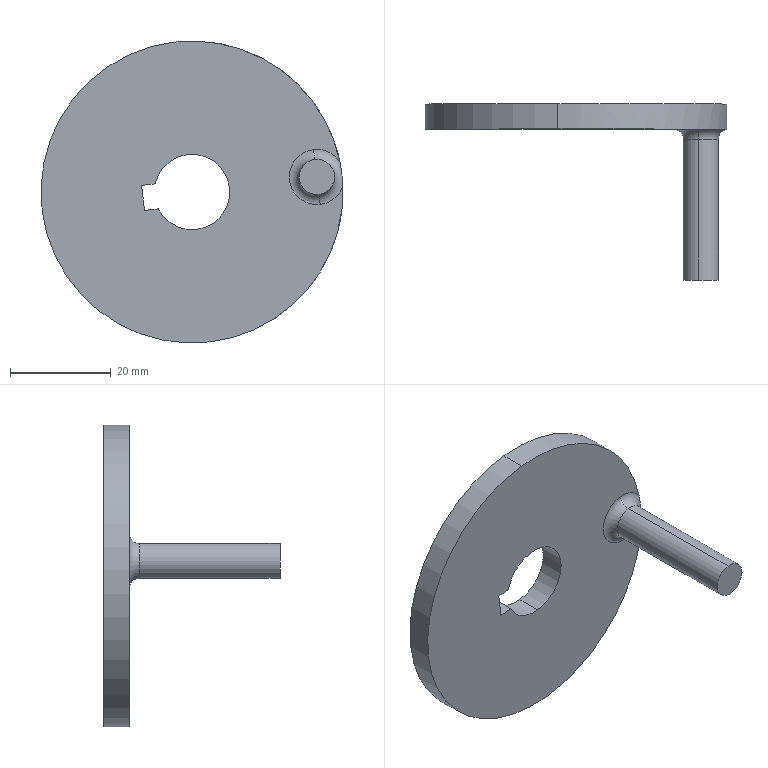Component | SolidWorks | CrankshaftOne-2_NewCrank-1 | 1 solid | 15 faces | box 60 x 35 x 60 mm | volume 14368 mm3 | cylinder 7 | plane 6 | torus 2 | commonest cylinder face diameters 15 x3 7 x2 60 x2 | material AISI 1045 Steel, Cold Drawn
STEP:
#1=COLOUR_RGB('',0.7922,0.8196,0.9333);
#2=FILL_AREA_STYLE_COLOUR('',#1);
#3=FILL_AREA_STYLE('',(#2));
#4=SURFACE_STYLE_FILL_AREA(#3);
#5=SURFACE_SIDE_STYLE('',(#4));
#6=SURFACE_STYLE_USAGE(.BOTH.,#5);
#7=PRESENTATION_STYLE_ASSIGNMENT((#6));
#8=CARTESIAN_POINT('',(1.263,0.7191,-6.574));
#9=VERTEX_POINT('',#8);
#10=CARTESIAN_POINT('',(1.23,0.7191,-6.301));
#11=VERTEX_POINT('',#10);
#12=CARTESIAN_POINT('',(1.247,0.7191,-6.438));
#13=DIRECTION('',(-0.,-1.,-0.));
#14=DIRECTION('',(0.1196,0.,-0.9928));
#15=AXIS2_PLACEMENT_3D('',#12,#13,#14);
#16=CIRCLE('',#15,0.1378);
#17=EDGE_CURVE('',#9,#11,#16,.T.);
#18=ORIENTED_EDGE('',*,*,#17,.F.);
#19=CARTESIAN_POINT('',(1.263,1.821,-6.574));
#20=VERTEX_POINT('',#19);
#21=CARTESIAN_POINT('',(1.263,0.7191,-6.574));
#22=DIRECTION('',(0.,1.,0.));
#23=VECTOR('',#22,39.37);
#24=LINE('',#21,#23);
#25=EDGE_CURVE('',#9,#20,#24,.T.);
#26=ORIENTED_EDGE('',*,*,#25,.T.);
#27=CARTESIAN_POINT('',(1.23,1.821,-6.301));
#28=VERTEX_POINT('',#27);
#29=CARTESIAN_POINT('',(1.247,1.821,-6.438));
#30=DIRECTION('',(-0.,-1.,-0.));
#31=DIRECTION('',(-0.1196,0.,0.9928));
#32=AXIS2_PLACEMENT_3D('',#29,#30,#31);
#33=CIRCLE('',#32,0.1378);
#34=EDGE_CURVE('',#20,#28,#33,.T.);
#35=ORIENTED_EDGE('',*,*,#34,.T.);
#36=CARTESIAN_POINT('',(1.23,0.7191,-6.301));
#37=DIRECTION('',(0.,1.,0.));
#38=VECTOR('',#37,39.37);
#39=LINE('',#36,#38);
#40=EDGE_CURVE('',#11,#28,#39,.T.);
#41=ORIENTED_EDGE('',*,*,#40,.F.);
#42=EDGE_LOOP('',(#18,#26,#35,#41));
#43=FACE_OUTER_BOUND('',#42,.T.);
#44=CARTESIAN_POINT('',(1.247,0.7191,-6.438));
#45=DIRECTION('',(0.,1.,0.));
#46=DIRECTION('',(-0.1196,0.,0.9928));
#47=AXIS2_PLACEMENT_3D('',#44,#45,#46);
#48=CYLINDRICAL_SURFACE('',#47,0.1378);
#49=ADVANCED_FACE('',(#43),#48,.T.);
#50=CARTESIAN_POINT('',(0.1282,2.097,-5.383));
#51=VERTEX_POINT('',#50);
#52=CARTESIAN_POINT('',(0.4108,2.097,-7.728));
#53=VERTEX_POINT('',#52);
#54=CARTESIAN_POINT('',(0.2695,2.097,-6.555));
#55=DIRECTION('',(0.,1.,0.));
#56=DIRECTION('',(-0.1196,0.,0.9928));
#57=AXIS2_PLACEMENT_3D('',#54,#55,#56);
#58=CIRCLE('',#57,1.181);
#59=EDGE_CURVE('',#51,#53,#58,.T.);
#60=ORIENTED_EDGE('',*,*,#59,.F.);
#61=CARTESIAN_POINT('',(0.1282,1.9,-5.383));
#62=VERTEX_POINT('',#61);
#63=CARTESIAN_POINT('',(0.1282,2.097,-5.383));
#64=DIRECTION('',(-0.,-1.,-0.));
#65=VECTOR('',#64,39.37);
#66=LINE('',#63,#65);
#67=EDGE_CURVE('',#51,#62,#66,.T.);
#68=ORIENTED_EDGE('',*,*,#67,.T.);
#69=CARTESIAN_POINT('',(1.426,1.9,-6.317));
#70=VERTEX_POINT('',#69);
#71=CARTESIAN_POINT('',(0.2695,1.9,-6.555));
#72=DIRECTION('',(0.,1.,0.));
#73=DIRECTION('',(-0.1196,0.,0.9928));
#74=AXIS2_PLACEMENT_3D('',#71,#72,#73);
#75=CIRCLE('',#74,1.181);
#76=EDGE_CURVE('',#62,#70,#75,.T.);
#77=ORIENTED_EDGE('',*,*,#76,.T.);
#78=CARTESIAN_POINT('',(1.45,1.9,-6.513));
#79=VERTEX_POINT('',#78);
#80=CARTESIAN_POINT('',(1.426,1.9,-6.317));
#81=CARTESIAN_POINT('',(1.43,1.9,-6.333));
#82=CARTESIAN_POINT('',(1.433,1.9,-6.349));
#83=CARTESIAN_POINT('',(1.438,1.898,-6.381));
#84=CARTESIAN_POINT('',(1.44,1.898,-6.398));
#85=CARTESIAN_POINT('',(1.444,1.898,-6.43));
#86=CARTESIAN_POINT('',(1.446,1.898,-6.447));
#87=CARTESIAN_POINT('',(1.448,1.9,-6.48));
#88=CARTESIAN_POINT('',(1.449,1.9,-6.496));
#89=CARTESIAN_POINT('',(1.45,1.9,-6.513));
#90=B_SPLINE_CURVE_WITH_KNOTS('',3,(#80,#81,#82,#83,#84,#85,#86,#87,#88,#89),.UNSPECIFIED.,.F.,.F.,(4,2,2,2,4),(0.,0.001254,0.002508,0.003762,0.005016),.UNSPECIFIED.);
#91=EDGE_CURVE('',#70,#79,#90,.T.);
#92=ORIENTED_EDGE('',*,*,#91,.T.);
#93=CARTESIAN_POINT('',(0.4108,1.9,-7.728));
#94=VERTEX_POINT('',#93);
#95=CARTESIAN_POINT('',(0.2695,1.9,-6.555));
#96=DIRECTION('',(0.,1.,0.));
#97=DIRECTION('',(-0.1196,0.,0.9928));
#98=AXIS2_PLACEMENT_3D('',#95,#96,#97);
#99=CIRCLE('',#98,1.181);
#100=EDGE_CURVE('',#79,#94,#99,.T.);
#101=ORIENTED_EDGE('',*,*,#100,.T.);
#102=CARTESIAN_POINT('',(0.4108,2.097,-7.728));
#103=DIRECTION('',(-0.,-1.,-0.));
#104=VECTOR('',#103,39.37);
#105=LINE('',#102,#104);
#106=EDGE_CURVE('',#53,#94,#105,.T.);
#107=ORIENTED_EDGE('',*,*,#106,.F.);
#108=EDGE_LOOP('',(#60,#68,#77,#92,#101,#107));
#109=FACE_OUTER_BOUND('',#108,.T.);
#110=CARTESIAN_POINT('',(0.2695,2.097,-6.555));
#111=DIRECTION('',(-0.,-1.,-0.));
#112=DIRECTION('',(0.1196,0.,-0.9928));
#113=AXIS2_PLACEMENT_3D('',#110,#111,#112);
#114=CYLINDRICAL_SURFACE('',#113,1.181);
#115=ADVANCED_FACE('',(#109),#114,.T.);
#116=CARTESIAN_POINT('',(-0.01865,2.097,-6.491));
#117=VERTEX_POINT('',#116);
#118=CARTESIAN_POINT('',(0.2342,2.097,-6.262));
#119=VERTEX_POINT('',#118);
#120=CARTESIAN_POINT('',(0.2695,2.097,-6.555));
#121=DIRECTION('',(0.,1.,0.));
#122=DIRECTION('',(-0.1196,0.,0.9928));
#123=AXIS2_PLACEMENT_3D('',#120,#121,#122);
#124=CIRCLE('',#123,0.2953);
#125=EDGE_CURVE('',#117,#119,#124,.T.);
#126=ORIENTED_EDGE('',*,*,#125,.T.);
#127=CARTESIAN_POINT('',(0.2342,1.9,-6.262));
#128=VERTEX_POINT('',#127);
#129=CARTESIAN_POINT('',(0.2342,2.097,-6.262));
#130=DIRECTION('',(-0.,-1.,-0.));
#131=VECTOR('',#130,39.37);
#132=LINE('',#129,#131);
#133=EDGE_CURVE('',#119,#128,#132,.T.);
#134=ORIENTED_EDGE('',*,*,#133,.T.);
#135=CARTESIAN_POINT('',(-0.01865,1.9,-6.491));
#136=VERTEX_POINT('',#135);
#137=CARTESIAN_POINT('',(0.2695,1.9,-6.555));
#138=DIRECTION('',(0.,1.,0.));
#139=DIRECTION('',(-0.1196,0.,0.9928));
#140=AXIS2_PLACEMENT_3D('',#137,#138,#139);
#141=CIRCLE('',#140,0.2953);
#142=EDGE_CURVE('',#136,#128,#141,.T.);
#143=ORIENTED_EDGE('',*,*,#142,.F.);
#144=CARTESIAN_POINT('',(-0.01865,2.097,-6.491));
#145=DIRECTION('',(-0.,-1.,-0.));
#146=VECTOR('',#145,39.37);
#147=LINE('',#144,#146);
#148=EDGE_CURVE('',#117,#136,#147,.T.);
#149=ORIENTED_EDGE('',*,*,#148,.F.);
#150=EDGE_LOOP('',(#126,#134,#143,#149));
#151=FACE_OUTER_BOUND('',#150,.T.);
#152=CARTESIAN_POINT('',(0.2695,2.097,-6.555));
#153=DIRECTION('',(-0.,-1.,-0.));
#154=DIRECTION('',(0.1196,0.,-0.9928));
#155=AXIS2_PLACEMENT_3D('',#152,#153,#154);
#156=CYLINDRICAL_SURFACE('',#155,0.2953);
#157=ADVANCED_FACE('',(#151),#156,.F.);
#158=ORIENTED_EDGE('',*,*,#133,.F.);
#159=CARTESIAN_POINT('',(0.3048,2.097,-6.849));
#160=VERTEX_POINT('',#159);
#161=CARTESIAN_POINT('',(0.2695,2.097,-6.555));
#162=DIRECTION('',(0.,1.,0.));
#163=DIRECTION('',(-0.1196,0.,0.9928));
#164=AXIS2_PLACEMENT_3D('',#161,#162,#163);
#165=CIRCLE('',#164,0.2953);
#166=EDGE_CURVE('',#119,#160,#165,.T.);
#167=ORIENTED_EDGE('',*,*,#166,.T.);
#168=CARTESIAN_POINT('',(0.3048,1.9,-6.849));
#169=VERTEX_POINT('',#168);
#170=CARTESIAN_POINT('',(0.3048,2.097,-6.849));
#171=DIRECTION('',(-0.,-1.,-0.));
#172=VECTOR('',#171,39.37);
#173=LINE('',#170,#172);
#174=EDGE_CURVE('',#160,#169,#173,.T.);
#175=ORIENTED_EDGE('',*,*,#174,.T.);
#176=CARTESIAN_POINT('',(0.2695,1.9,-6.555));
#177=DIRECTION('',(0.,1.,0.));
#178=DIRECTION('',(-0.1196,0.,0.9928));
#179=AXIS2_PLACEMENT_3D('',#176,#177,#178);
#180=CIRCLE('',#179,0.2953);
#181=EDGE_CURVE('',#128,#169,#180,.T.);
#182=ORIENTED_EDGE('',*,*,#181,.F.);
#183=EDGE_LOOP('',(#158,#167,#175,#182));
#184=FACE_OUTER_BOUND('',#183,.T.);
#185=CARTESIAN_POINT('',(0.2695,2.097,-6.555));
#186=DIRECTION('',(-0.,-1.,-0.));
#187=DIRECTION('',(0.1196,0.,-0.9928));
#188=AXIS2_PLACEMENT_3D('',#185,#186,#187);
#189=CYLINDRICAL_SURFACE('',#188,0.2953);
#190=ADVANCED_FACE('',(#184),#189,.F.);
#191=CARTESIAN_POINT('',(1.273,1.9,-6.653));
#192=VERTEX_POINT('',#191);
#193=CARTESIAN_POINT('',(1.221,1.9,-6.223));
#194=VERTEX_POINT('',#193);
#195=CARTESIAN_POINT('',(1.247,1.9,-6.438));
#196=DIRECTION('',(0.,1.,0.));
#197=DIRECTION('',(-0.1196,0.,0.9928));
#198=AXIS2_PLACEMENT_3D('',#195,#196,#197);
#199=CIRCLE('',#198,0.2165);
#200=EDGE_CURVE('',#192,#194,#199,.T.);
#201=ORIENTED_EDGE('',*,*,#200,.F.);
#202=CARTESIAN_POINT('',(1.273,1.821,-6.653));
#203=DIRECTION('',(0.9928,-0.,0.1196));
#204=DIRECTION('',(0.1196,0.,-0.9928));
#205=AXIS2_PLACEMENT_3D('',#202,#203,#204);
#206=CIRCLE('',#205,0.07874);
#207=EDGE_CURVE('',#192,#20,#206,.T.);
#208=ORIENTED_EDGE('',*,*,#207,.T.);
#209=CARTESIAN_POINT('',(1.247,1.821,-6.438));
#210=DIRECTION('',(-0.,-1.,-0.));
#211=DIRECTION('',(-0.1196,0.,0.9928));
#212=AXIS2_PLACEMENT_3D('',#209,#210,#211);
#213=CIRCLE('',#212,0.1378);
#214=EDGE_CURVE('',#28,#20,#213,.T.);
#215=ORIENTED_EDGE('',*,*,#214,.F.);
#216=CARTESIAN_POINT('',(1.221,1.821,-6.223));
#217=DIRECTION('',(-0.9928,0.,-0.1196));
#218=DIRECTION('',(-0.1196,0.,0.9928));
#219=AXIS2_PLACEMENT_3D('',#216,#217,#218);
#220=CIRCLE('',#219,0.07874);
#221=EDGE_CURVE('',#194,#28,#220,.T.);
#222=ORIENTED_EDGE('',*,*,#221,.F.);
#223=EDGE_LOOP('',(#201,#208,#215,#222));
#224=FACE_OUTER_BOUND('',#223,.T.);
#225=CARTESIAN_POINT('',(1.247,1.821,-6.438));
#226=DIRECTION('',(0.,1.,0.));
#227=DIRECTION('',(-0.1196,-0.,0.9928));
#228=AXIS2_PLACEMENT_3D('',#225,#226,#227);
#229=TOROIDAL_SURFACE('',#228,0.2165,0.07874);
#230=ADVANCED_FACE('',(#224),#229,.F.);
#231=ORIENTED_EDGE('',*,*,#207,.F.);
#232=CARTESIAN_POINT('',(1.247,1.9,-6.438));
#233=DIRECTION('',(0.,1.,0.));
#234=DIRECTION('',(-0.1196,0.,0.9928));
#235=AXIS2_PLACEMENT_3D('',#232,#233,#234);
#236=CIRCLE('',#235,0.2165);
#237=EDGE_CURVE('',#79,#192,#236,.T.);
#238=ORIENTED_EDGE('',*,*,#237,.F.);
#239=ORIENTED_EDGE('',*,*,#91,.F.);
#240=CARTESIAN_POINT('',(1.247,1.9,-6.438));
#241=DIRECTION('',(0.,1.,0.));
#242=DIRECTION('',(-0.1196,0.,0.9928));
#243=AXIS2_PLACEMENT_3D('',#240,#241,#242);
#244=CIRCLE('',#243,0.2165);
#245=EDGE_CURVE('',#194,#70,#244,.T.);
#246=ORIENTED_EDGE('',*,*,#245,.F.);
#247=ORIENTED_EDGE('',*,*,#221,.T.);
#248=ORIENTED_EDGE('',*,*,#34,.F.);
#249=EDGE_LOOP('',(#231,#238,#239,#246,#247,#248));
#250=FACE_OUTER_BOUND('',#249,.T.);
#251=CARTESIAN_POINT('',(1.247,1.821,-6.438));
#252=DIRECTION('',(0.,1.,0.));
#253=DIRECTION('',(-0.1196,-0.,0.9928));
#254=AXIS2_PLACEMENT_3D('',#251,#252,#253);
#255=TOROIDAL_SURFACE('',#254,0.2165,0.07874);
#256=ADVANCED_FACE('',(#250),#255,.F.);
#257=CARTESIAN_POINT('',(-0.1018,1.9,-6.699));
#258=VERTEX_POINT('',#257);
#259=CARTESIAN_POINT('',(-0.1253,1.9,-6.504));
#260=VERTEX_POINT('',#259);
#261=CARTESIAN_POINT('',(-0.1135,1.9,-6.602));
#262=DIRECTION('',(-0.1196,-0.,0.9928));
#263=VECTOR('',#262,39.37);
#264=LINE('',#261,#263);
#265=EDGE_CURVE('',#258,#260,#264,.T.);
#266=ORIENTED_EDGE('',*,*,#265,.T.);
#267=CARTESIAN_POINT('',(0.2577,1.9,-6.458));
#268=DIRECTION('',(0.9928,-0.,0.1196));
#269=VECTOR('',#268,39.37);
#270=LINE('',#267,#269);
#271=EDGE_CURVE('',#260,#136,#270,.T.);
#272=ORIENTED_EDGE('',*,*,#271,.T.);
#273=ORIENTED_EDGE('',*,*,#142,.T.);
#274=ORIENTED_EDGE('',*,*,#181,.T.);
#275=CARTESIAN_POINT('',(0.004901,1.9,-6.686));
#276=VERTEX_POINT('',#275);
#277=CARTESIAN_POINT('',(0.2695,1.9,-6.555));
#278=DIRECTION('',(0.,1.,0.));
#279=DIRECTION('',(-0.1196,0.,0.9928));
#280=AXIS2_PLACEMENT_3D('',#277,#278,#279);
#281=CIRCLE('',#280,0.2953);
#282=EDGE_CURVE('',#169,#276,#281,.T.);
#283=ORIENTED_EDGE('',*,*,#282,.T.);
#284=CARTESIAN_POINT('',(0.2813,1.9,-6.653));
#285=DIRECTION('',(-0.9928,0.,-0.1196));
#286=VECTOR('',#285,39.37);
#287=LINE('',#284,#286);
#288=EDGE_CURVE('',#276,#258,#287,.T.);
#289=ORIENTED_EDGE('',*,*,#288,.T.);
#290=EDGE_LOOP('',(#266,#272,#273,#274,#283,#289));
#291=FACE_BOUND('',#290,.T.);
#292=ORIENTED_EDGE('',*,*,#100,.F.);
#293=ORIENTED_EDGE('',*,*,#237,.T.);
#294=ORIENTED_EDGE('',*,*,#200,.T.);
#295=ORIENTED_EDGE('',*,*,#245,.T.);
#296=ORIENTED_EDGE('',*,*,#76,.F.);
#297=CARTESIAN_POINT('',(0.2695,1.9,-6.555));
#298=DIRECTION('',(0.,1.,0.));
#299=DIRECTION('',(-0.1196,0.,0.9928));
#300=AXIS2_PLACEMENT_3D('',#297,#298,#299);
#301=CIRCLE('',#300,1.181);
#302=EDGE_CURVE('',#94,#62,#301,.T.);
#303=ORIENTED_EDGE('',*,*,#302,.F.);
#304=EDGE_LOOP('',(#292,#293,#294,#295,#296,#303));
#305=FACE_OUTER_BOUND('',#304,.T.);
#306=CARTESIAN_POINT('',(0.2695,1.9,-6.555));
#307=DIRECTION('',(0.,1.,0.));
#308=DIRECTION('',(-0.1196,-0.,0.9928));
#309=AXIS2_PLACEMENT_3D('',#306,#307,#308);
#310=PLANE('',#309);
#311=ADVANCED_FACE('',(#291,#305),#310,.F.);
#312=ORIENTED_EDGE('',*,*,#174,.F.);
#313=CARTESIAN_POINT('',(0.004901,2.097,-6.686));
#314=VERTEX_POINT('',#313);
#315=CARTESIAN_POINT('',(0.2695,2.097,-6.555));
#316=DIRECTION('',(0.,1.,0.));
#317=DIRECTION('',(-0.1196,0.,0.9928));
#318=AXIS2_PLACEMENT_3D('',#315,#316,#317);
#319=CIRCLE('',#318,0.2953);
#320=EDGE_CURVE('',#160,#314,#319,.T.);
#321=ORIENTED_EDGE('',*,*,#320,.T.);
#322=CARTESIAN_POINT('',(0.004901,2.097,-6.686));
#323=DIRECTION('',(0.,1.,0.));
#324=VECTOR('',#323,39.37);
#325=LINE('',#322,#324);
#326=EDGE_CURVE('',#276,#314,#325,.T.);
#327=ORIENTED_EDGE('',*,*,#326,.F.);
#328=ORIENTED_EDGE('',*,*,#282,.F.);
#329=EDGE_LOOP('',(#312,#321,#327,#328));
#330=FACE_OUTER_BOUND('',#329,.T.);
#331=CARTESIAN_POINT('',(0.2695,2.097,-6.555));
#332=DIRECTION('',(-0.,-1.,-0.));
#333=DIRECTION('',(0.1196,0.,-0.9928));
#334=AXIS2_PLACEMENT_3D('',#331,#332,#333);
#335=CYLINDRICAL_SURFACE('',#334,0.2953);
#336=ADVANCED_FACE('',(#330),#335,.F.);
#337=ORIENTED_EDGE('',*,*,#67,.F.);
#338=CARTESIAN_POINT('',(0.2695,2.097,-6.555));
#339=DIRECTION('',(0.,1.,0.));
#340=DIRECTION('',(-0.1196,0.,0.9928));
#341=AXIS2_PLACEMENT_3D('',#338,#339,#340);
#342=CIRCLE('',#341,1.181);
#343=EDGE_CURVE('',#53,#51,#342,.T.);
#344=ORIENTED_EDGE('',*,*,#343,.F.);
#345=ORIENTED_EDGE('',*,*,#106,.T.);
#346=ORIENTED_EDGE('',*,*,#302,.T.);
#347=EDGE_LOOP('',(#337,#344,#345,#346));
#348=FACE_OUTER_BOUND('',#347,.T.);
#349=CARTESIAN_POINT('',(0.2695,2.097,-6.555));
#350=DIRECTION('',(-0.,-1.,-0.));
#351=DIRECTION('',(0.1196,0.,-0.9928));
#352=AXIS2_PLACEMENT_3D('',#349,#350,#351);
#353=CYLINDRICAL_SURFACE('',#352,1.181);
#354=ADVANCED_FACE('',(#348),#353,.T.);
#355=CARTESIAN_POINT('',(-0.1253,2.097,-6.504));
#356=VERTEX_POINT('',#355);
#357=CARTESIAN_POINT('',(0.2577,2.097,-6.458));
#358=DIRECTION('',(0.9928,-0.,0.1196));
#359=VECTOR('',#358,39.37);
#360=LINE('',#357,#359);
#361=EDGE_CURVE('',#356,#117,#360,.T.);
#362=ORIENTED_EDGE('',*,*,#361,.F.);
#363=CARTESIAN_POINT('',(-0.1018,2.097,-6.699));
#364=VERTEX_POINT('',#363);
#365=CARTESIAN_POINT('',(-0.1018,2.097,-6.699));
#366=DIRECTION('',(-0.1196,-0.,0.9928));
#367=VECTOR('',#366,39.37);
#368=LINE('',#365,#367);
#369=EDGE_CURVE('',#364,#356,#368,.T.);
#370=ORIENTED_EDGE('',*,*,#369,.F.);
#371=CARTESIAN_POINT('',(0.2813,2.097,-6.653));
#372=DIRECTION('',(-0.9928,0.,-0.1196));
#373=VECTOR('',#372,39.37);
#374=LINE('',#371,#373);
#375=EDGE_CURVE('',#314,#364,#374,.T.);
#376=ORIENTED_EDGE('',*,*,#375,.F.);
#377=ORIENTED_EDGE('',*,*,#320,.F.);
#378=ORIENTED_EDGE('',*,*,#166,.F.);
#379=ORIENTED_EDGE('',*,*,#125,.F.);
#380=EDGE_LOOP('',(#362,#370,#376,#377,#378,#379));
#381=FACE_BOUND('',#380,.T.);
#382=ORIENTED_EDGE('',*,*,#343,.T.);
#383=ORIENTED_EDGE('',*,*,#59,.T.);
#384=EDGE_LOOP('',(#382,#383));
#385=FACE_OUTER_BOUND('',#384,.T.);
#386=CARTESIAN_POINT('',(0.2695,2.097,-6.555));
#387=DIRECTION('',(0.,1.,0.));
#388=DIRECTION('',(-0.1196,-0.,0.9928));
#389=AXIS2_PLACEMENT_3D('',#386,#387,#388);
#390=PLANE('',#389);
#391=ADVANCED_FACE('',(#381,#385),#390,.T.);
#392=CARTESIAN_POINT('',(-0.1018,1.703,-6.699));
#393=DIRECTION('',(0.,1.,0.));
#394=VECTOR('',#393,39.37);
#395=LINE('',#392,#394);
#396=EDGE_CURVE('',#258,#364,#395,.T.);
#397=ORIENTED_EDGE('',*,*,#396,.T.);
#398=ORIENTED_EDGE('',*,*,#369,.T.);
#399=CARTESIAN_POINT('',(-0.1253,1.703,-6.504));
#400=DIRECTION('',(0.,1.,0.));
#401=VECTOR('',#400,39.37);
#402=LINE('',#399,#401);
#403=EDGE_CURVE('',#260,#356,#402,.T.);
#404=ORIENTED_EDGE('',*,*,#403,.F.);
#405=ORIENTED_EDGE('',*,*,#265,.F.);
#406=EDGE_LOOP('',(#397,#398,#404,#405));
#407=FACE_OUTER_BOUND('',#406,.T.);
#408=CARTESIAN_POINT('',(-0.1018,1.703,-6.699));
#409=DIRECTION('',(-0.9928,0.,-0.1196));
#410=DIRECTION('',(-0.,-1.,-0.));
#411=AXIS2_PLACEMENT_3D('',#408,#409,#410);
#412=PLANE('',#411);
#413=ADVANCED_FACE('',(#407),#412,.F.);
#414=ORIENTED_EDGE('',*,*,#148,.T.);
#415=ORIENTED_EDGE('',*,*,#271,.F.);
#416=ORIENTED_EDGE('',*,*,#403,.T.);
#417=ORIENTED_EDGE('',*,*,#361,.T.);
#418=EDGE_LOOP('',(#414,#415,#416,#417));
#419=FACE_OUTER_BOUND('',#418,.T.);
#420=CARTESIAN_POINT('',(0.2577,1.703,-6.458));
#421=DIRECTION('',(-0.1196,-0.,0.9928));
#422=DIRECTION('',(0.9928,-0.,0.1196));
#423=AXIS2_PLACEMENT_3D('',#420,#421,#422);
#424=PLANE('',#423);
#425=ADVANCED_FACE('',(#419),#424,.F.);
#426=ORIENTED_EDGE('',*,*,#326,.T.);
#427=ORIENTED_EDGE('',*,*,#375,.T.);
#428=ORIENTED_EDGE('',*,*,#396,.F.);
#429=ORIENTED_EDGE('',*,*,#288,.F.);
#430=EDGE_LOOP('',(#426,#427,#428,#429));
#431=FACE_OUTER_BOUND('',#430,.T.);
#432=CARTESIAN_POINT('',(0.2813,1.703,-6.653));
#433=DIRECTION('',(0.1196,0.,-0.9928));
#434=DIRECTION('',(-0.9928,0.,-0.1196));
#435=AXIS2_PLACEMENT_3D('',#432,#433,#434);
#436=PLANE('',#435);
#437=ADVANCED_FACE('',(#431),#436,.F.);
#438=ORIENTED_EDGE('',*,*,#25,.F.);
#439=CARTESIAN_POINT('',(1.247,0.7191,-6.438));
#440=DIRECTION('',(-0.,-1.,-0.));
#441=DIRECTION('',(0.1196,0.,-0.9928));
#442=AXIS2_PLACEMENT_3D('',#439,#440,#441);
#443=CIRCLE('',#442,0.1378);
#444=EDGE_CURVE('',#11,#9,#443,.T.);
#445=ORIENTED_EDGE('',*,*,#444,.F.);
#446=ORIENTED_EDGE('',*,*,#40,.T.);
#447=ORIENTED_EDGE('',*,*,#214,.T.);
#448=EDGE_LOOP('',(#438,#445,#446,#447));
#449=FACE_OUTER_BOUND('',#448,.T.);
#450=CARTESIAN_POINT('',(1.247,0.7191,-6.438));
#451=DIRECTION('',(0.,1.,0.));
#452=DIRECTION('',(-0.1196,0.,0.9928));
#453=AXIS2_PLACEMENT_3D('',#450,#451,#452);
#454=CYLINDRICAL_SURFACE('',#453,0.1378);
#455=ADVANCED_FACE('',(#449),#454,.T.);
#456=ORIENTED_EDGE('',*,*,#444,.T.);
#457=ORIENTED_EDGE('',*,*,#17,.T.);
#458=EDGE_LOOP('',(#456,#457));
#459=FACE_OUTER_BOUND('',#458,.T.);
#460=CARTESIAN_POINT('',(1.247,0.7191,-6.438));
#461=DIRECTION('',(-0.,-1.,-0.));
#462=DIRECTION('',(0.1196,0.,-0.9928));
#463=AXIS2_PLACEMENT_3D('',#460,#461,#462);
#464=PLANE('',#463);
#465=ADVANCED_FACE('',(#459),#464,.T.);
#466=CLOSED_SHELL('',(#49,#115,#157,#190,#230,#256,#311,#336,#354,#391,#413,#425,#437,#455,#465));
#467=MANIFOLD_SOLID_BREP('',#466);
#468=STYLED_ITEM('',(#7),#467);
#469=(LENGTH_UNIT()NAMED_UNIT(*)SI_UNIT($,.METRE.));
#470=LENGTH_MEASURE_WITH_UNIT(LENGTH_MEASURE(0.0254),#469);
#471=DIMENSIONAL_EXPONENTS(1.,0.,0.,0.,0.,0.,0.);
#472=(CONVERSION_BASED_UNIT('',#470)LENGTH_UNIT()NAMED_UNIT(#471));
#473=UNCERTAINTY_MEASURE_WITH_UNIT(LENGTH_MEASURE(0.00001),#472,'','');
#474=(NAMED_UNIT(*)PLANE_ANGLE_UNIT()SI_UNIT($,.RADIAN.));
#475=(NAMED_UNIT(*)SI_UNIT($,.STERADIAN.)SOLID_ANGLE_UNIT());
#476=(GEOMETRIC_REPRESENTATION_CONTEXT(3)GLOBAL_UNCERTAINTY_ASSIGNED_CONTEXT((#473))GLOBAL_UNIT_ASSIGNED_CONTEXT((#472,#474,#475))REPRESENTATION_CONTEXT('',''));
#477=MECHANICAL_DESIGN_GEOMETRIC_PRESENTATION_REPRESENTATION('',(#468),#476);
#478=CARTESIAN_POINT('',(0.,0.,0.));
#479=DIRECTION('',(0.,0.,1.));
#480=DIRECTION('',(1.,0.,0.));
#481=AXIS2_PLACEMENT_3D('',#478,#479,#480);
#482=(LENGTH_UNIT()NAMED_UNIT(*)SI_UNIT($,.METRE.));
#483=LENGTH_MEASURE_WITH_UNIT(LENGTH_MEASURE(0.0254),#482);
#484=DIMENSIONAL_EXPONENTS(1.,0.,0.,0.,0.,0.,0.);
#485=(CONVERSION_BASED_UNIT('',#483)LENGTH_UNIT()NAMED_UNIT(#484));
#486=UNCERTAINTY_MEASURE_WITH_UNIT(LENGTH_MEASURE(0.00001),#485,'','');
#487=(NAMED_UNIT(*)PLANE_ANGLE_UNIT()SI_UNIT($,.RADIAN.));
#488=(NAMED_UNIT(*)SI_UNIT($,.STERADIAN.)SOLID_ANGLE_UNIT());
#489=(GEOMETRIC_REPRESENTATION_CONTEXT(3)GLOBAL_UNCERTAINTY_ASSIGNED_CONTEXT((#486))GLOBAL_UNIT_ASSIGNED_CONTEXT((#485,#487,#488))REPRESENTATION_CONTEXT('',''));
#490=ADVANCED_BREP_SHAPE_REPRESENTATION('',(#467,#481),#489);
#491=PRESENTATION_LAYER_ASSIGNMENT('','',(#468));